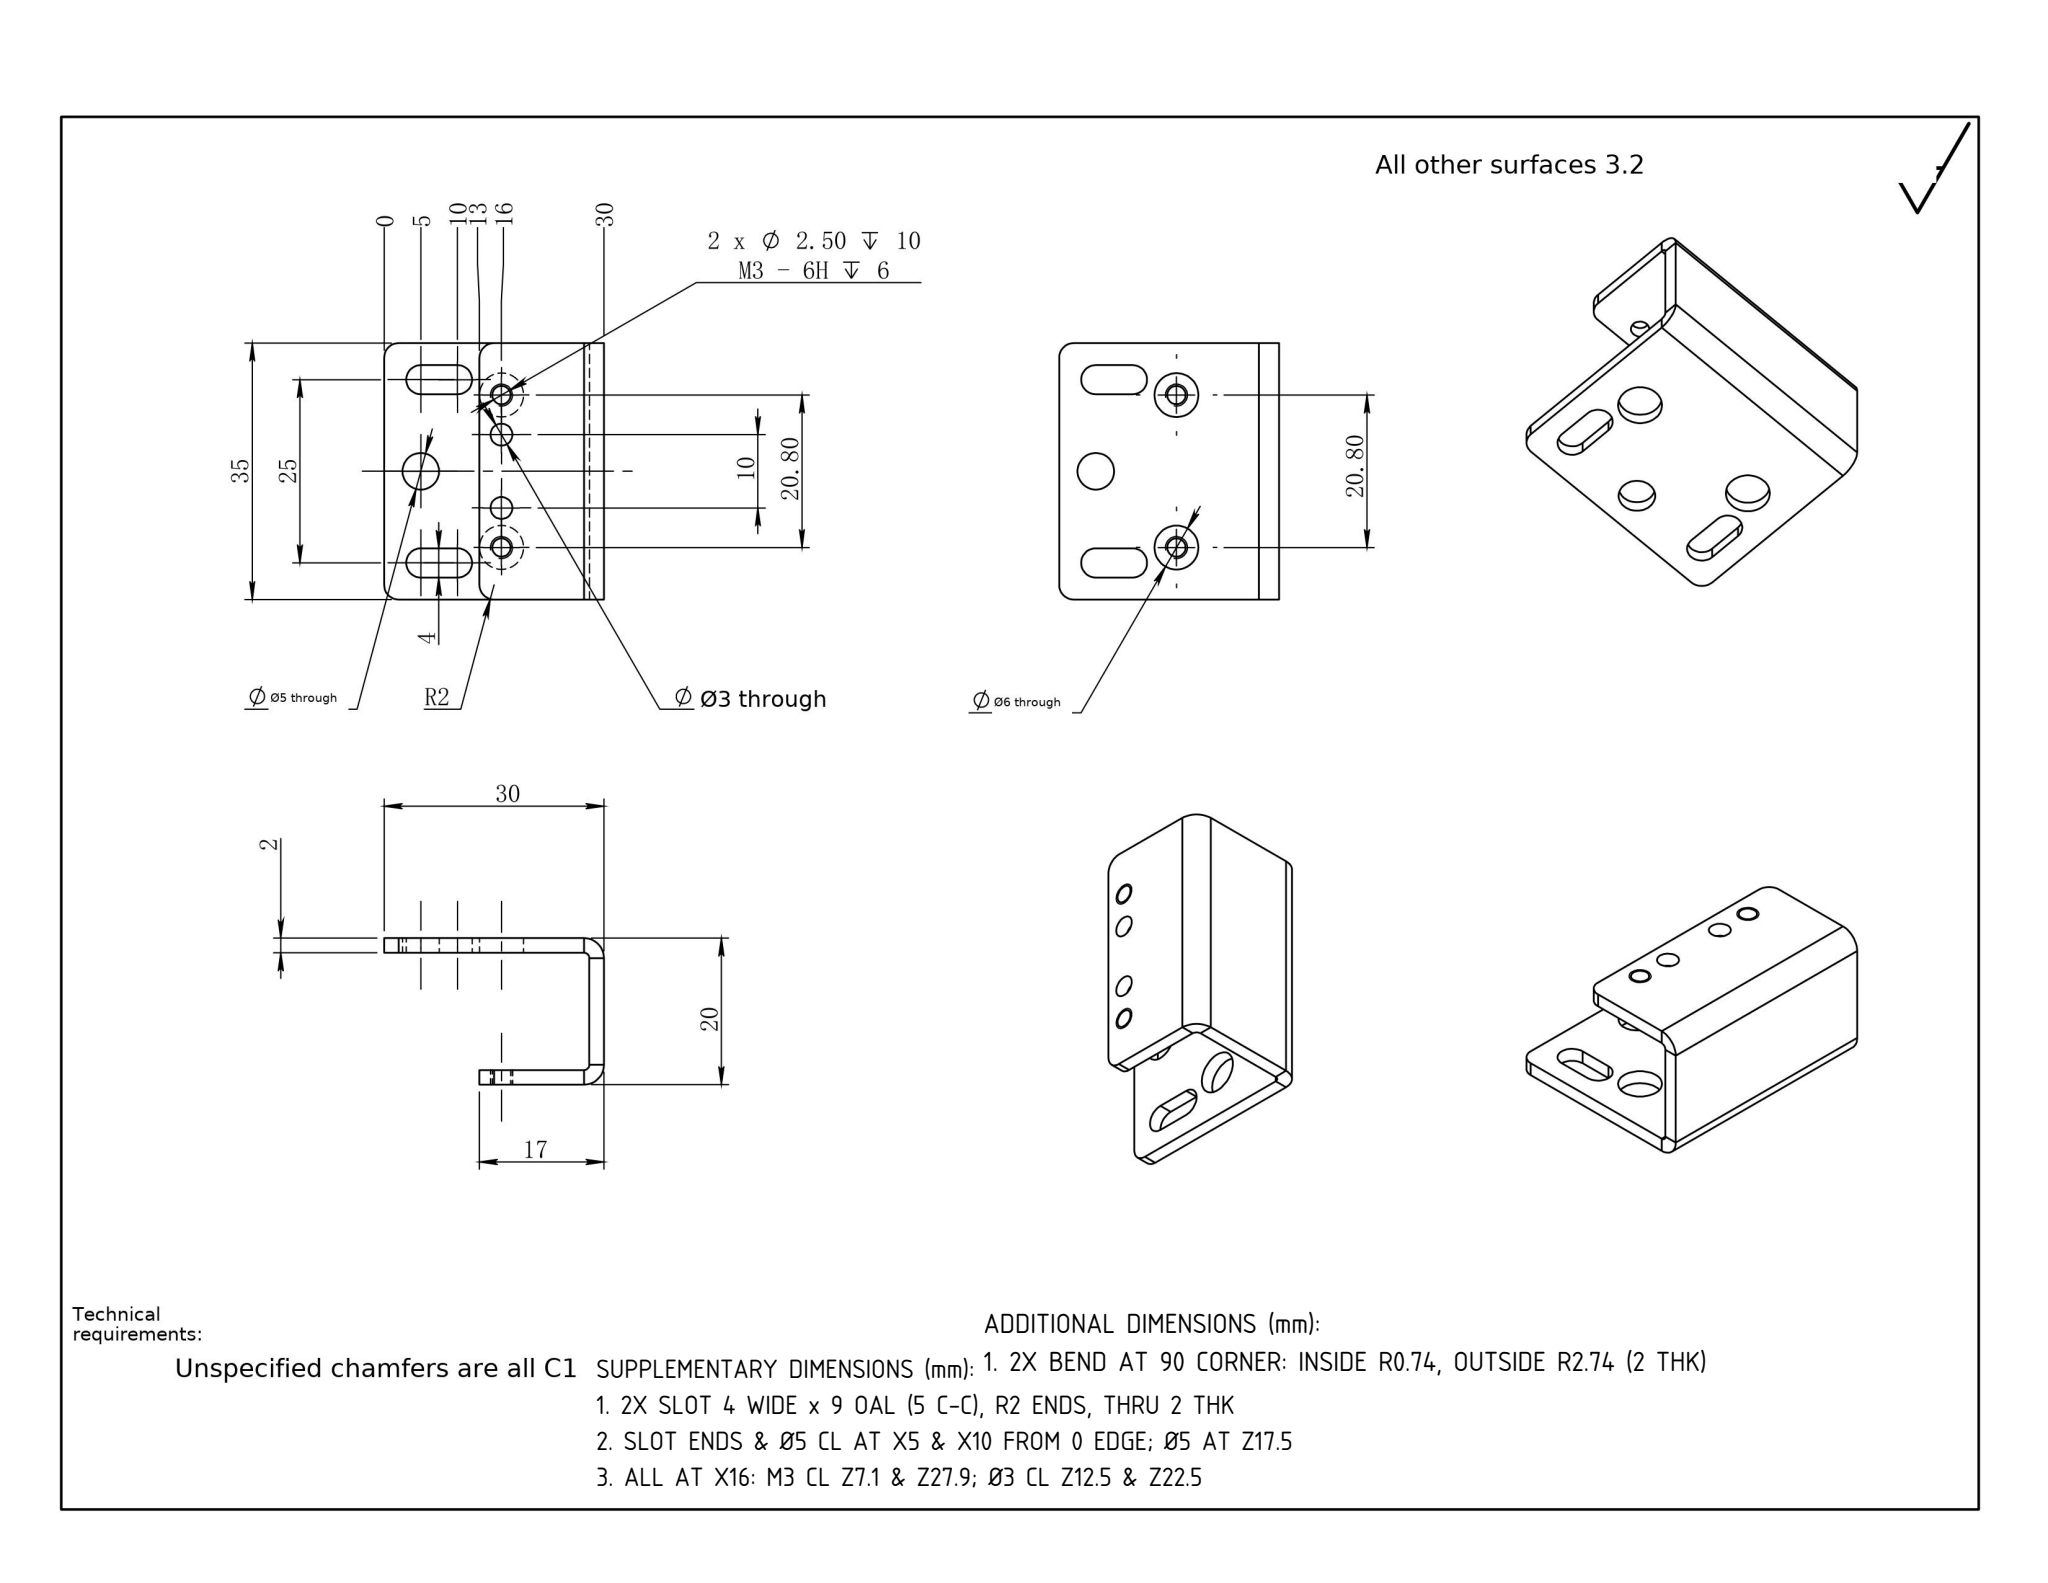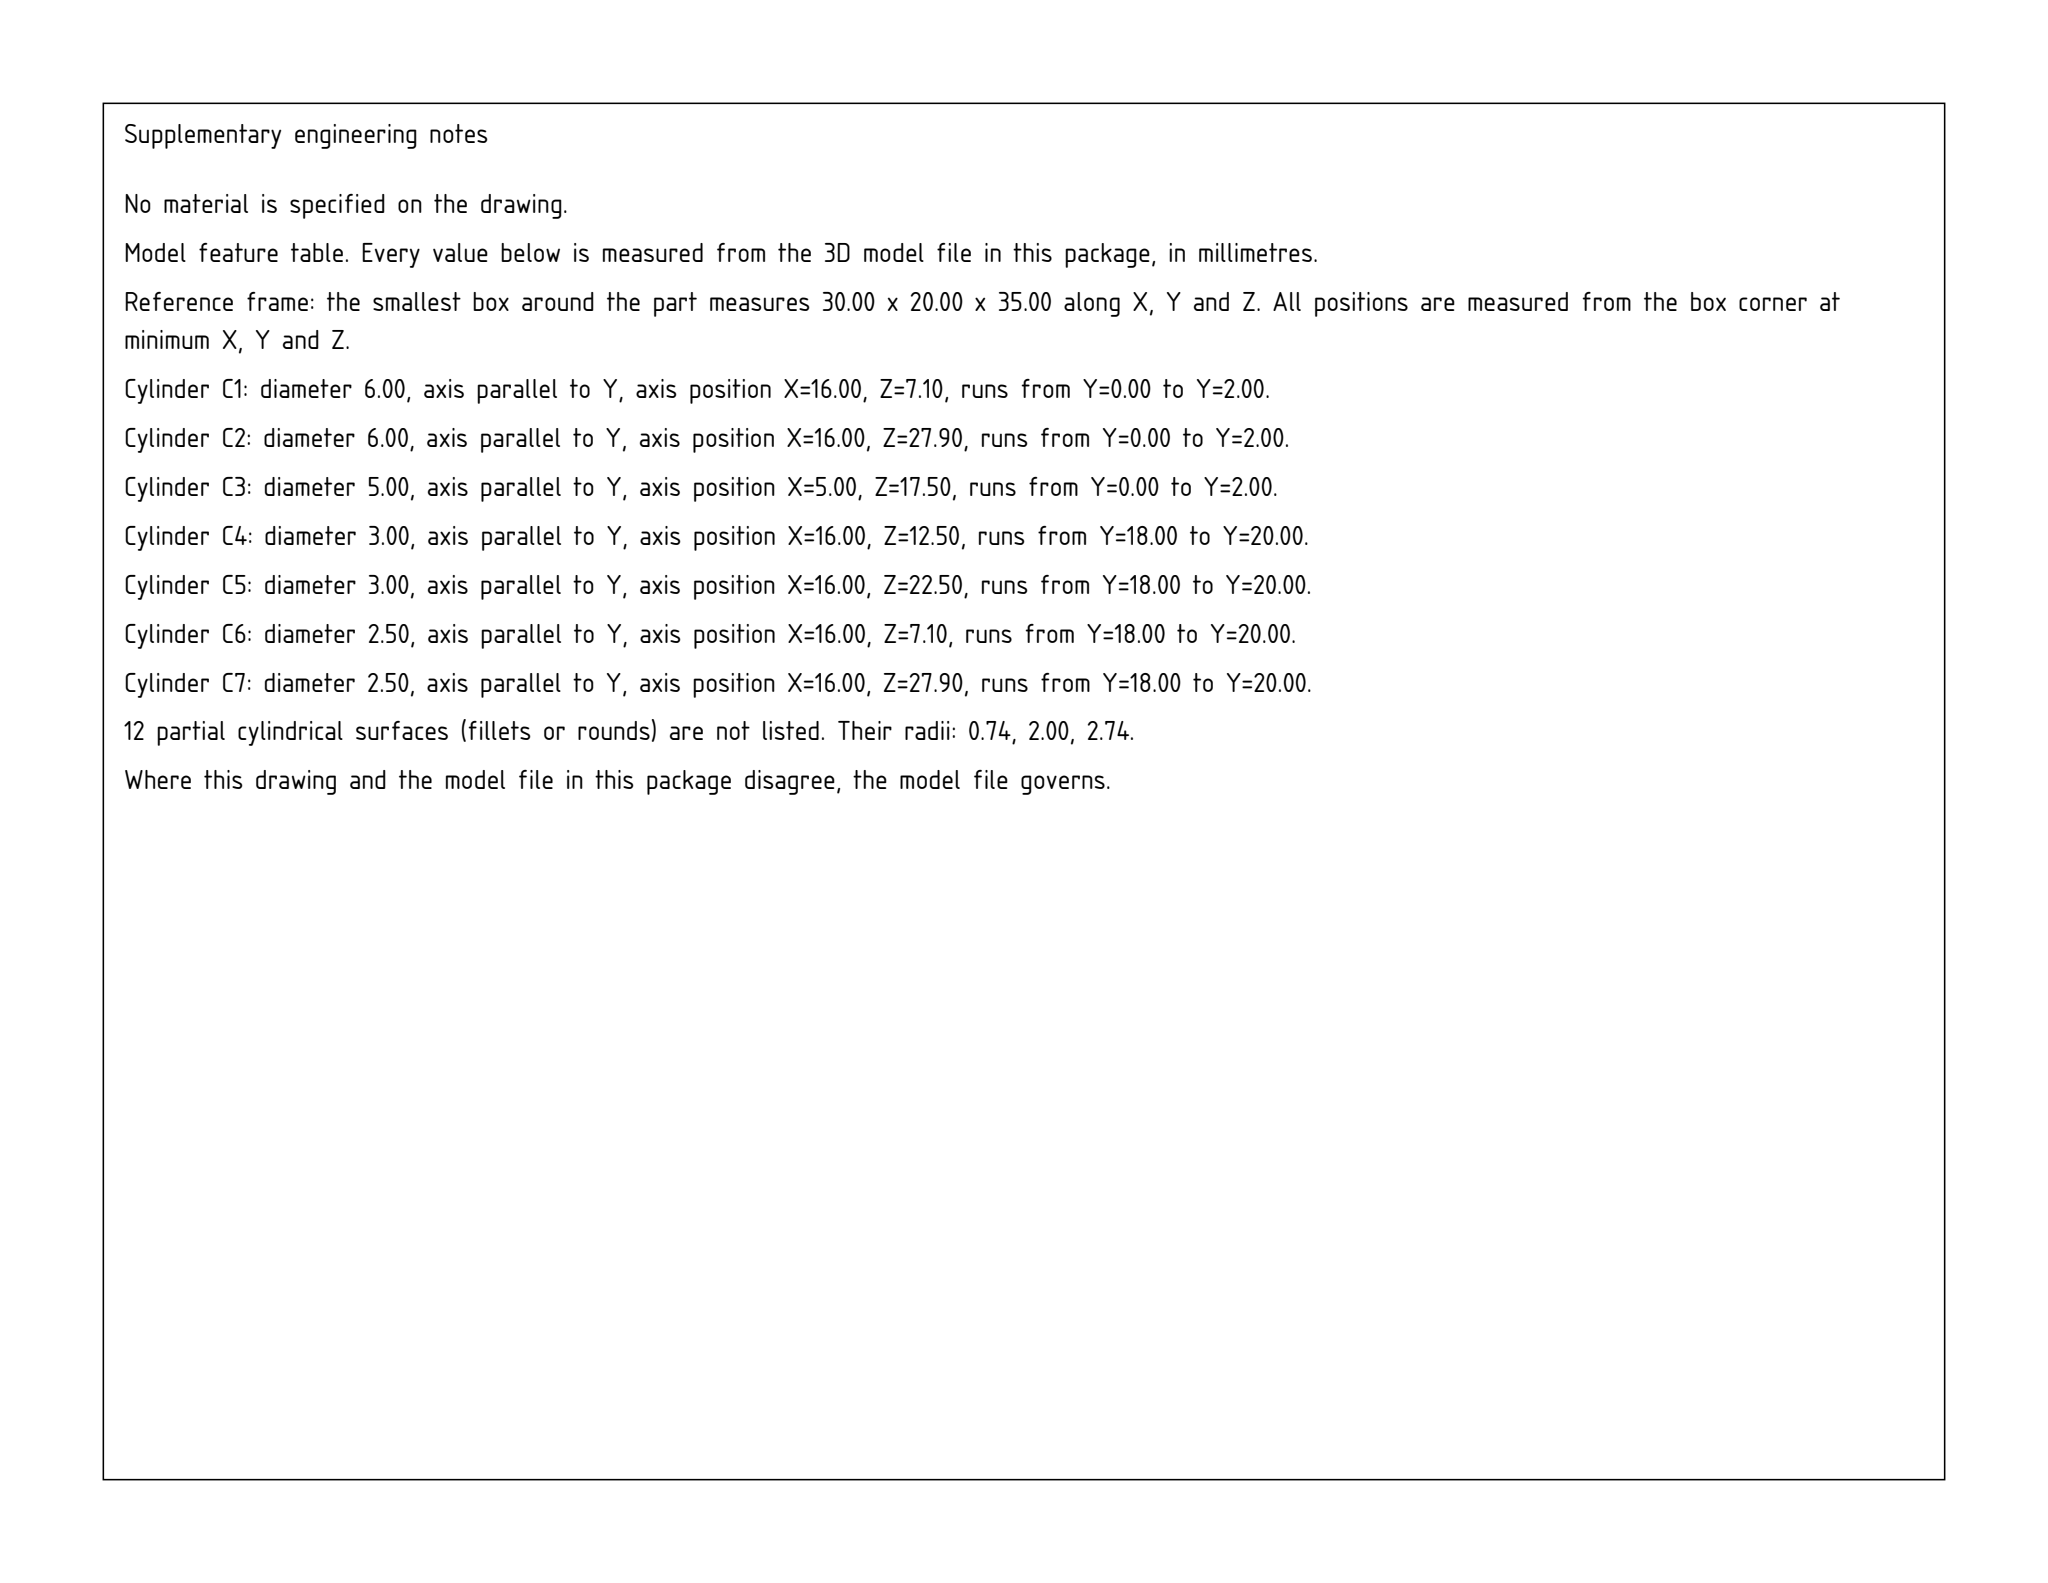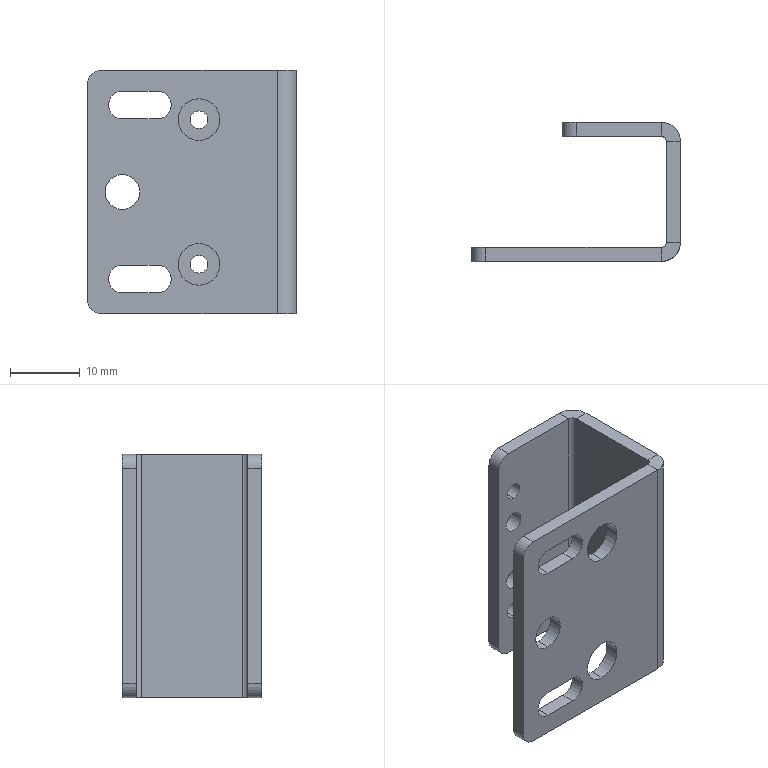Part | SolidWorks | mm | 1 solid | 48 faces | box 30 x 20 x 35 mm | volume 3968 mm3 | cylinder 26 | plane 22 | commonest cylinder face diameters 4 x8 6 x4 3 x4 2.5 x4 5 x2 5.473 x2 1.473 x2